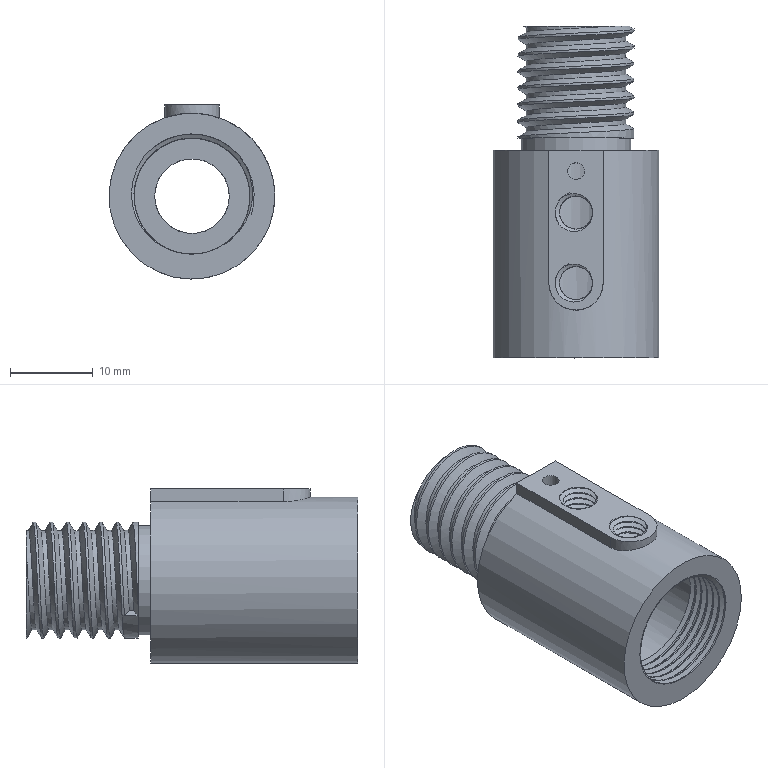Component | NX | VALVE_BODY | 1 solid | 41 faces | volume 5861 mm3 | cylinder 21 | plane 12 | spline 8 | commonest cylinder face diameters 14 x8 4 x3 5 x3 20 x1 13.25 x1 12 x1 6.545 x1 9 x1